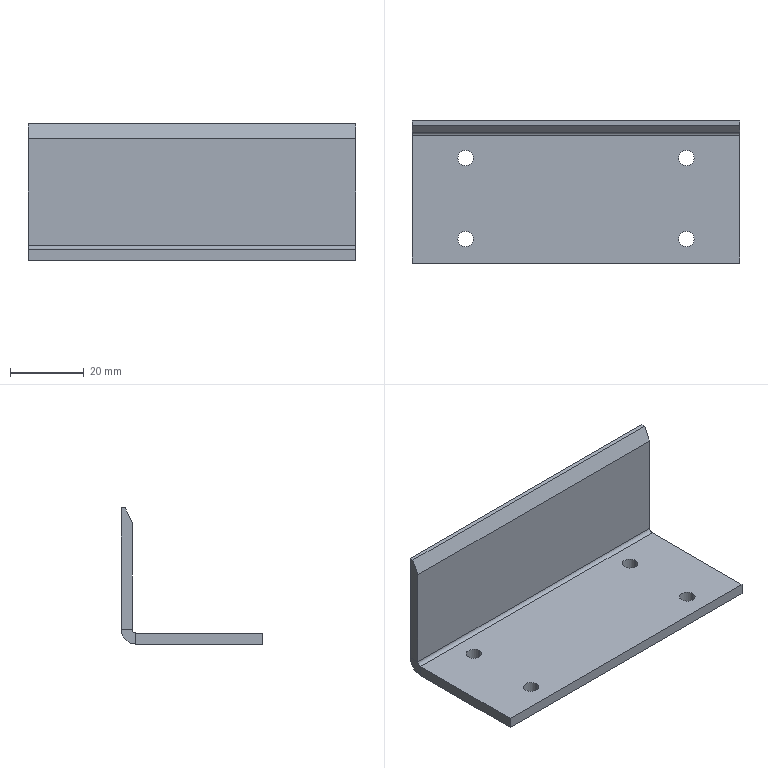Component | SolidWorks | AA-1_TransitionPlate-1 | 1 solid | 23 faces | box 89 x 38.51 x 37 mm | volume 18576 mm3 | plane 13 | cylinder 10 | commonest cylinder face diameters 4.2 x8 2 x1 8 x1
STEP:
#1=COLOUR_RGB('',0.7922,0.8196,0.9333);
#2=FILL_AREA_STYLE_COLOUR('',#1);
#3=FILL_AREA_STYLE('',(#2));
#4=SURFACE_STYLE_FILL_AREA(#3);
#5=SURFACE_SIDE_STYLE('',(#4));
#6=SURFACE_STYLE_USAGE(.BOTH.,#5);
#7=PRESENTATION_STYLE_ASSIGNMENT((#6));
#8=CARTESIAN_POINT('',(-18.558,-12.235,44.862));
#9=VERTEX_POINT('',#8);
#10=CARTESIAN_POINT('',(-18.393,-12.235,44.862));
#11=VERTEX_POINT('',#10);
#12=CARTESIAN_POINT('',(-18.475,-12.235,44.862));
#13=DIRECTION('',(-0.,0.,1.));
#14=DIRECTION('',(1.,0.,0.));
#15=AXIS2_PLACEMENT_3D('',#12,#13,#14);
#16=CIRCLE('',#15,0.08268);
#17=EDGE_CURVE('',#9,#11,#16,.T.);
#18=ORIENTED_EDGE('',*,*,#17,.F.);
#19=CARTESIAN_POINT('',(-18.558,-12.235,44.98));
#20=VERTEX_POINT('',#19);
#21=CARTESIAN_POINT('',(-18.558,-12.235,44.98));
#22=DIRECTION('',(-0.,0.,1.));
#23=VECTOR('',#22,39.37);
#24=LINE('',#21,#23);
#25=EDGE_CURVE('',#9,#20,#24,.T.);
#26=ORIENTED_EDGE('',*,*,#25,.T.);
#27=CARTESIAN_POINT('',(-18.393,-12.235,44.98));
#28=VERTEX_POINT('',#27);
#29=CARTESIAN_POINT('',(-18.475,-12.235,44.98));
#30=DIRECTION('',(-0.,0.,1.));
#31=DIRECTION('',(1.,0.,0.));
#32=AXIS2_PLACEMENT_3D('',#29,#30,#31);
#33=CIRCLE('',#32,0.08268);
#34=EDGE_CURVE('',#20,#28,#33,.T.);
#35=ORIENTED_EDGE('',*,*,#34,.T.);
#36=CARTESIAN_POINT('',(-18.393,-12.235,44.98));
#37=DIRECTION('',(-0.,0.,1.));
#38=VECTOR('',#37,39.37);
#39=LINE('',#36,#38);
#40=EDGE_CURVE('',#11,#28,#39,.T.);
#41=ORIENTED_EDGE('',*,*,#40,.F.);
#42=EDGE_LOOP('',(#18,#26,#35,#41));
#43=FACE_OUTER_BOUND('',#42,.T.);
#44=CARTESIAN_POINT('',(-18.475,-12.235,44.98));
#45=DIRECTION('',(-0.,0.,1.));
#46=DIRECTION('',(1.,0.,0.));
#47=AXIS2_PLACEMENT_3D('',#44,#45,#46);
#48=CYLINDRICAL_SURFACE('',#47,0.08268);
#49=ADVANCED_FACE('',(#43),#48,.F.);
#50=CARTESIAN_POINT('',(-16.196,-12.235,44.862));
#51=VERTEX_POINT('',#50);
#52=CARTESIAN_POINT('',(-16.03,-12.235,44.862));
#53=VERTEX_POINT('',#52);
#54=CARTESIAN_POINT('',(-16.113,-12.235,44.862));
#55=DIRECTION('',(-0.,0.,1.));
#56=DIRECTION('',(1.,0.,0.));
#57=AXIS2_PLACEMENT_3D('',#54,#55,#56);
#58=CIRCLE('',#57,0.08268);
#59=EDGE_CURVE('',#51,#53,#58,.T.);
#60=ORIENTED_EDGE('',*,*,#59,.F.);
#61=CARTESIAN_POINT('',(-16.196,-12.235,44.98));
#62=VERTEX_POINT('',#61);
#63=CARTESIAN_POINT('',(-16.196,-12.235,44.98));
#64=DIRECTION('',(-0.,0.,1.));
#65=VECTOR('',#64,39.37);
#66=LINE('',#63,#65);
#67=EDGE_CURVE('',#51,#62,#66,.T.);
#68=ORIENTED_EDGE('',*,*,#67,.T.);
#69=CARTESIAN_POINT('',(-16.03,-12.235,44.98));
#70=VERTEX_POINT('',#69);
#71=CARTESIAN_POINT('',(-16.113,-12.235,44.98));
#72=DIRECTION('',(-0.,0.,1.));
#73=DIRECTION('',(1.,0.,0.));
#74=AXIS2_PLACEMENT_3D('',#71,#72,#73);
#75=CIRCLE('',#74,0.08268);
#76=EDGE_CURVE('',#62,#70,#75,.T.);
#77=ORIENTED_EDGE('',*,*,#76,.T.);
#78=CARTESIAN_POINT('',(-16.03,-12.235,44.98));
#79=DIRECTION('',(-0.,0.,1.));
#80=VECTOR('',#79,39.37);
#81=LINE('',#78,#80);
#82=EDGE_CURVE('',#53,#70,#81,.T.);
#83=ORIENTED_EDGE('',*,*,#82,.F.);
#84=EDGE_LOOP('',(#60,#68,#77,#83));
#85=FACE_OUTER_BOUND('',#84,.T.);
#86=CARTESIAN_POINT('',(-16.113,-12.235,44.98));
#87=DIRECTION('',(-0.,0.,1.));
#88=DIRECTION('',(1.,0.,0.));
#89=AXIS2_PLACEMENT_3D('',#86,#87,#88);
#90=CYLINDRICAL_SURFACE('',#89,0.08268);
#91=ADVANCED_FACE('',(#85),#90,.F.);
#92=CARTESIAN_POINT('',(-16.196,-13.102,44.862));
#93=VERTEX_POINT('',#92);
#94=CARTESIAN_POINT('',(-16.03,-13.102,44.862));
#95=VERTEX_POINT('',#94);
#96=CARTESIAN_POINT('',(-16.113,-13.102,44.862));
#97=DIRECTION('',(-0.,0.,1.));
#98=DIRECTION('',(1.,0.,0.));
#99=AXIS2_PLACEMENT_3D('',#96,#97,#98);
#100=CIRCLE('',#99,0.08268);
#101=EDGE_CURVE('',#93,#95,#100,.T.);
#102=ORIENTED_EDGE('',*,*,#101,.F.);
#103=CARTESIAN_POINT('',(-16.196,-13.102,44.98));
#104=VERTEX_POINT('',#103);
#105=CARTESIAN_POINT('',(-16.196,-13.102,44.98));
#106=DIRECTION('',(-0.,0.,1.));
#107=VECTOR('',#106,39.37);
#108=LINE('',#105,#107);
#109=EDGE_CURVE('',#93,#104,#108,.T.);
#110=ORIENTED_EDGE('',*,*,#109,.T.);
#111=CARTESIAN_POINT('',(-16.03,-13.102,44.98));
#112=VERTEX_POINT('',#111);
#113=CARTESIAN_POINT('',(-16.113,-13.102,44.98));
#114=DIRECTION('',(-0.,0.,1.));
#115=DIRECTION('',(1.,0.,0.));
#116=AXIS2_PLACEMENT_3D('',#113,#114,#115);
#117=CIRCLE('',#116,0.08268);
#118=EDGE_CURVE('',#104,#112,#117,.T.);
#119=ORIENTED_EDGE('',*,*,#118,.T.);
#120=CARTESIAN_POINT('',(-16.03,-13.102,44.98));
#121=DIRECTION('',(-0.,0.,1.));
#122=VECTOR('',#121,39.37);
#123=LINE('',#120,#122);
#124=EDGE_CURVE('',#95,#112,#123,.T.);
#125=ORIENTED_EDGE('',*,*,#124,.F.);
#126=EDGE_LOOP('',(#102,#110,#119,#125));
#127=FACE_OUTER_BOUND('',#126,.T.);
#128=CARTESIAN_POINT('',(-16.113,-13.102,44.98));
#129=DIRECTION('',(-0.,0.,1.));
#130=DIRECTION('',(1.,0.,0.));
#131=AXIS2_PLACEMENT_3D('',#128,#129,#130);
#132=CYLINDRICAL_SURFACE('',#131,0.08268);
#133=ADVANCED_FACE('',(#127),#132,.F.);
#134=CARTESIAN_POINT('',(-18.558,-13.102,44.862));
#135=VERTEX_POINT('',#134);
#136=CARTESIAN_POINT('',(-18.393,-13.102,44.862));
#137=VERTEX_POINT('',#136);
#138=CARTESIAN_POINT('',(-18.475,-13.102,44.862));
#139=DIRECTION('',(-0.,0.,1.));
#140=DIRECTION('',(1.,0.,0.));
#141=AXIS2_PLACEMENT_3D('',#138,#139,#140);
#142=CIRCLE('',#141,0.08268);
#143=EDGE_CURVE('',#135,#137,#142,.T.);
#144=ORIENTED_EDGE('',*,*,#143,.F.);
#145=CARTESIAN_POINT('',(-18.558,-13.102,44.98));
#146=VERTEX_POINT('',#145);
#147=CARTESIAN_POINT('',(-18.558,-13.102,44.98));
#148=DIRECTION('',(-0.,0.,1.));
#149=VECTOR('',#148,39.37);
#150=LINE('',#147,#149);
#151=EDGE_CURVE('',#135,#146,#150,.T.);
#152=ORIENTED_EDGE('',*,*,#151,.T.);
#153=CARTESIAN_POINT('',(-18.393,-13.102,44.98));
#154=VERTEX_POINT('',#153);
#155=CARTESIAN_POINT('',(-18.475,-13.102,44.98));
#156=DIRECTION('',(-0.,0.,1.));
#157=DIRECTION('',(1.,0.,0.));
#158=AXIS2_PLACEMENT_3D('',#155,#156,#157);
#159=CIRCLE('',#158,0.08268);
#160=EDGE_CURVE('',#146,#154,#159,.T.);
#161=ORIENTED_EDGE('',*,*,#160,.T.);
#162=CARTESIAN_POINT('',(-18.393,-13.102,44.98));
#163=DIRECTION('',(-0.,0.,1.));
#164=VECTOR('',#163,39.37);
#165=LINE('',#162,#164);
#166=EDGE_CURVE('',#137,#154,#165,.T.);
#167=ORIENTED_EDGE('',*,*,#166,.F.);
#168=EDGE_LOOP('',(#144,#152,#161,#167));
#169=FACE_OUTER_BOUND('',#168,.T.);
#170=CARTESIAN_POINT('',(-18.475,-13.102,44.98));
#171=DIRECTION('',(-0.,0.,1.));
#172=DIRECTION('',(1.,0.,0.));
#173=AXIS2_PLACEMENT_3D('',#170,#171,#172);
#174=CYLINDRICAL_SURFACE('',#173,0.08268);
#175=ADVANCED_FACE('',(#169),#174,.F.);
#176=CARTESIAN_POINT('',(-15.542,-11.959,45.02));
#177=VERTEX_POINT('',#176);
#178=CARTESIAN_POINT('',(-15.542,-11.841,45.02));
#179=VERTEX_POINT('',#178);
#180=CARTESIAN_POINT('',(-15.542,-11.959,45.02));
#181=DIRECTION('',(-0.,1.,-0.));
#182=VECTOR('',#181,39.37);
#183=LINE('',#180,#182);
#184=EDGE_CURVE('',#177,#179,#183,.T.);
#185=ORIENTED_EDGE('',*,*,#184,.F.);
#186=CARTESIAN_POINT('',(-15.542,-11.999,44.98));
#187=VERTEX_POINT('',#186);
#188=CARTESIAN_POINT('',(-15.542,-11.999,45.02));
#189=DIRECTION('',(1.,0.,0.));
#190=DIRECTION('',(0.,0.,1.));
#191=AXIS2_PLACEMENT_3D('',#188,#189,#190);
#192=CIRCLE('',#191,0.03937);
#193=EDGE_CURVE('',#187,#177,#192,.T.);
#194=ORIENTED_EDGE('',*,*,#193,.F.);
#195=CARTESIAN_POINT('',(-15.542,-11.999,44.862));
#196=VERTEX_POINT('',#195);
#197=CARTESIAN_POINT('',(-15.542,-11.999,44.862));
#198=DIRECTION('',(-0.,0.,1.));
#199=VECTOR('',#198,39.37);
#200=LINE('',#197,#199);
#201=EDGE_CURVE('',#196,#187,#200,.T.);
#202=ORIENTED_EDGE('',*,*,#201,.F.);
#203=CARTESIAN_POINT('',(-15.542,-11.999,45.02));
#204=DIRECTION('',(1.,0.,0.));
#205=DIRECTION('',(0.,0.,-1.));
#206=AXIS2_PLACEMENT_3D('',#203,#204,#205);
#207=CIRCLE('',#206,0.1575);
#208=EDGE_CURVE('',#196,#179,#207,.T.);
#209=ORIENTED_EDGE('',*,*,#208,.T.);
#210=EDGE_LOOP('',(#185,#194,#202,#209));
#211=FACE_OUTER_BOUND('',#210,.T.);
#212=CARTESIAN_POINT('',(-15.542,-11.959,45.02));
#213=DIRECTION('',(1.,0.,0.));
#214=DIRECTION('',(0.,-0.,-1.));
#215=AXIS2_PLACEMENT_3D('',#212,#213,#214);
#216=PLANE('',#215);
#217=ADVANCED_FACE('',(#211),#216,.T.);
#218=CARTESIAN_POINT('',(-15.542,-11.886,46.319));
#219=VERTEX_POINT('',#218);
#220=CARTESIAN_POINT('',(-15.542,-11.841,46.319));
#221=VERTEX_POINT('',#220);
#222=CARTESIAN_POINT('',(-15.542,-11.959,46.319));
#223=DIRECTION('',(-0.,1.,-0.));
#224=VECTOR('',#223,39.37);
#225=LINE('',#222,#224);
#226=EDGE_CURVE('',#219,#221,#225,.T.);
#227=ORIENTED_EDGE('',*,*,#226,.F.);
#228=CARTESIAN_POINT('',(-15.542,-11.959,46.161));
#229=VERTEX_POINT('',#228);
#230=CARTESIAN_POINT('',(-15.542,-12.464,45.079));
#231=DIRECTION('',(0.,-0.4226,-0.9063));
#232=VECTOR('',#231,39.37);
#233=LINE('',#230,#232);
#234=EDGE_CURVE('',#219,#229,#233,.T.);
#235=ORIENTED_EDGE('',*,*,#234,.T.);
#236=CARTESIAN_POINT('',(-15.542,-11.959,44.98));
#237=DIRECTION('',(-0.,0.,1.));
#238=VECTOR('',#237,39.37);
#239=LINE('',#236,#238);
#240=EDGE_CURVE('',#177,#229,#239,.T.);
#241=ORIENTED_EDGE('',*,*,#240,.F.);
#242=ORIENTED_EDGE('',*,*,#184,.T.);
#243=CARTESIAN_POINT('',(-15.542,-11.841,44.98));
#244=DIRECTION('',(-0.,0.,1.));
#245=VECTOR('',#244,39.37);
#246=LINE('',#243,#245);
#247=EDGE_CURVE('',#179,#221,#246,.T.);
#248=ORIENTED_EDGE('',*,*,#247,.T.);
#249=EDGE_LOOP('',(#227,#235,#241,#242,#248));
#250=FACE_OUTER_BOUND('',#249,.T.);
#251=CARTESIAN_POINT('',(-15.542,-11.999,44.862));
#252=DIRECTION('',(1.,0.,0.));
#253=DIRECTION('',(0.,-0.,-1.));
#254=AXIS2_PLACEMENT_3D('',#251,#252,#253);
#255=PLANE('',#254);
#256=ADVANCED_FACE('',(#250),#255,.T.);
#257=CARTESIAN_POINT('',(-19.046,-11.999,44.98));
#258=VERTEX_POINT('',#257);
#259=CARTESIAN_POINT('',(-19.046,-11.999,44.862));
#260=VERTEX_POINT('',#259);
#261=CARTESIAN_POINT('',(-19.046,-11.999,44.98));
#262=DIRECTION('',(0.,-0.,-1.));
#263=VECTOR('',#262,39.37);
#264=LINE('',#261,#263);
#265=EDGE_CURVE('',#258,#260,#264,.T.);
#266=ORIENTED_EDGE('',*,*,#265,.F.);
#267=CARTESIAN_POINT('',(-19.046,-11.959,45.02));
#268=VERTEX_POINT('',#267);
#269=CARTESIAN_POINT('',(-19.046,-11.999,45.02));
#270=DIRECTION('',(1.,0.,0.));
#271=DIRECTION('',(0.,0.,1.));
#272=AXIS2_PLACEMENT_3D('',#269,#270,#271);
#273=CIRCLE('',#272,0.03937);
#274=EDGE_CURVE('',#258,#268,#273,.T.);
#275=ORIENTED_EDGE('',*,*,#274,.T.);
#276=CARTESIAN_POINT('',(-19.046,-11.841,45.02));
#277=VERTEX_POINT('',#276);
#278=CARTESIAN_POINT('',(-19.046,-11.841,45.02));
#279=DIRECTION('',(0.,-1.,0.));
#280=VECTOR('',#279,39.37);
#281=LINE('',#278,#280);
#282=EDGE_CURVE('',#277,#268,#281,.T.);
#283=ORIENTED_EDGE('',*,*,#282,.F.);
#284=CARTESIAN_POINT('',(-19.046,-11.999,45.02));
#285=DIRECTION('',(1.,0.,0.));
#286=DIRECTION('',(0.,0.,-1.));
#287=AXIS2_PLACEMENT_3D('',#284,#285,#286);
#288=CIRCLE('',#287,0.1575);
#289=EDGE_CURVE('',#260,#277,#288,.T.);
#290=ORIENTED_EDGE('',*,*,#289,.F.);
#291=EDGE_LOOP('',(#266,#275,#283,#290));
#292=FACE_OUTER_BOUND('',#291,.T.);
#293=CARTESIAN_POINT('',(-19.046,-11.999,44.98));
#294=DIRECTION('',(-1.,-0.,-0.));
#295=DIRECTION('',(-0.,0.,1.));
#296=AXIS2_PLACEMENT_3D('',#293,#294,#295);
#297=PLANE('',#296);
#298=ADVANCED_FACE('',(#292),#297,.T.);
#299=CARTESIAN_POINT('',(-19.046,-13.357,44.98));
#300=VERTEX_POINT('',#299);
#301=CARTESIAN_POINT('',(-19.046,-13.357,44.98));
#302=DIRECTION('',(-0.,1.,-0.));
#303=VECTOR('',#302,39.37);
#304=LINE('',#301,#303);
#305=EDGE_CURVE('',#300,#258,#304,.T.);
#306=ORIENTED_EDGE('',*,*,#305,.T.);
#307=ORIENTED_EDGE('',*,*,#265,.T.);
#308=CARTESIAN_POINT('',(-19.046,-13.357,44.862));
#309=VERTEX_POINT('',#308);
#310=CARTESIAN_POINT('',(-19.046,-13.357,44.862));
#311=DIRECTION('',(-0.,1.,-0.));
#312=VECTOR('',#311,39.37);
#313=LINE('',#310,#312);
#314=EDGE_CURVE('',#309,#260,#313,.T.);
#315=ORIENTED_EDGE('',*,*,#314,.F.);
#316=CARTESIAN_POINT('',(-19.046,-13.357,44.862));
#317=DIRECTION('',(-0.,0.,1.));
#318=VECTOR('',#317,39.37);
#319=LINE('',#316,#318);
#320=EDGE_CURVE('',#309,#300,#319,.T.);
#321=ORIENTED_EDGE('',*,*,#320,.T.);
#322=EDGE_LOOP('',(#306,#307,#315,#321));
#323=FACE_OUTER_BOUND('',#322,.T.);
#324=CARTESIAN_POINT('',(-19.046,-11.841,45.02));
#325=DIRECTION('',(-1.,-0.,-0.));
#326=DIRECTION('',(-0.,0.,1.));
#327=AXIS2_PLACEMENT_3D('',#324,#325,#326);
#328=PLANE('',#327);
#329=ADVANCED_FACE('',(#323),#328,.T.);
#330=CARTESIAN_POINT('',(-19.046,-11.841,46.319));
#331=VERTEX_POINT('',#330);
#332=CARTESIAN_POINT('',(-19.046,-11.841,44.98));
#333=DIRECTION('',(-0.,0.,1.));
#334=VECTOR('',#333,39.37);
#335=LINE('',#332,#334);
#336=EDGE_CURVE('',#277,#331,#335,.T.);
#337=ORIENTED_EDGE('',*,*,#336,.T.);
#338=CARTESIAN_POINT('',(-15.542,-11.841,46.319));
#339=DIRECTION('',(-1.,-0.,-0.));
#340=VECTOR('',#339,39.37);
#341=LINE('',#338,#340);
#342=EDGE_CURVE('',#221,#331,#341,.T.);
#343=ORIENTED_EDGE('',*,*,#342,.F.);
#344=ORIENTED_EDGE('',*,*,#247,.F.);
#345=CARTESIAN_POINT('',(-15.542,-11.841,45.02));
#346=DIRECTION('',(-1.,-0.,-0.));
#347=VECTOR('',#346,39.37);
#348=LINE('',#345,#347);
#349=EDGE_CURVE('',#179,#277,#348,.T.);
#350=ORIENTED_EDGE('',*,*,#349,.T.);
#351=EDGE_LOOP('',(#337,#343,#344,#350));
#352=FACE_OUTER_BOUND('',#351,.T.);
#353=CARTESIAN_POINT('',(-15.542,-11.841,44.98));
#354=DIRECTION('',(0.,-1.,0.));
#355=DIRECTION('',(-1.,-0.,-0.));
#356=AXIS2_PLACEMENT_3D('',#353,#354,#355);
#357=PLANE('',#356);
#358=ADVANCED_FACE('',(#352),#357,.F.);
#359=CARTESIAN_POINT('',(-19.046,-11.886,46.319));
#360=VERTEX_POINT('',#359);
#361=CARTESIAN_POINT('',(-19.046,-11.959,46.319));
#362=DIRECTION('',(-0.,1.,-0.));
#363=VECTOR('',#362,39.37);
#364=LINE('',#361,#363);
#365=EDGE_CURVE('',#360,#331,#364,.T.);
#366=ORIENTED_EDGE('',*,*,#365,.F.);
#367=CARTESIAN_POINT('',(-15.542,-11.886,46.319));
#368=DIRECTION('',(1.,0.,0.));
#369=VECTOR('',#368,39.37);
#370=LINE('',#367,#369);
#371=EDGE_CURVE('',#360,#219,#370,.T.);
#372=ORIENTED_EDGE('',*,*,#371,.T.);
#373=ORIENTED_EDGE('',*,*,#226,.T.);
#374=ORIENTED_EDGE('',*,*,#342,.T.);
#375=EDGE_LOOP('',(#366,#372,#373,#374));
#376=FACE_OUTER_BOUND('',#375,.T.);
#377=CARTESIAN_POINT('',(-15.542,-11.959,46.319));
#378=DIRECTION('',(-0.,0.,1.));
#379=DIRECTION('',(1.,0.,0.));
#380=AXIS2_PLACEMENT_3D('',#377,#378,#379);
#381=PLANE('',#380);
#382=ADVANCED_FACE('',(#376),#381,.T.);
#383=ORIENTED_EDGE('',*,*,#240,.T.);
#384=CARTESIAN_POINT('',(-19.046,-11.959,46.161));
#385=VERTEX_POINT('',#384);
#386=CARTESIAN_POINT('',(-15.542,-11.959,46.161));
#387=DIRECTION('',(-1.,-0.,-0.));
#388=VECTOR('',#387,39.37);
#389=LINE('',#386,#388);
#390=EDGE_CURVE('',#229,#385,#389,.T.);
#391=ORIENTED_EDGE('',*,*,#390,.T.);
#392=CARTESIAN_POINT('',(-19.046,-11.959,44.98));
#393=DIRECTION('',(-0.,0.,1.));
#394=VECTOR('',#393,39.37);
#395=LINE('',#392,#394);
#396=EDGE_CURVE('',#268,#385,#395,.T.);
#397=ORIENTED_EDGE('',*,*,#396,.F.);
#398=CARTESIAN_POINT('',(-15.542,-11.959,45.02));
#399=DIRECTION('',(-1.,-0.,-0.));
#400=VECTOR('',#399,39.37);
#401=LINE('',#398,#400);
#402=EDGE_CURVE('',#177,#268,#401,.T.);
#403=ORIENTED_EDGE('',*,*,#402,.F.);
#404=EDGE_LOOP('',(#383,#391,#397,#403));
#405=FACE_OUTER_BOUND('',#404,.T.);
#406=CARTESIAN_POINT('',(-15.542,-11.959,44.98));
#407=DIRECTION('',(0.,-1.,0.));
#408=DIRECTION('',(-1.,-0.,-0.));
#409=AXIS2_PLACEMENT_3D('',#406,#407,#408);
#410=PLANE('',#409);
#411=ADVANCED_FACE('',(#405),#410,.T.);
#412=ORIENTED_EDGE('',*,*,#274,.F.);
#413=CARTESIAN_POINT('',(-15.542,-11.999,44.98));
#414=DIRECTION('',(-1.,-0.,-0.));
#415=VECTOR('',#414,39.37);
#416=LINE('',#413,#415);
#417=EDGE_CURVE('',#187,#258,#416,.T.);
#418=ORIENTED_EDGE('',*,*,#417,.F.);
#419=ORIENTED_EDGE('',*,*,#193,.T.);
#420=ORIENTED_EDGE('',*,*,#402,.T.);
#421=EDGE_LOOP('',(#412,#418,#419,#420));
#422=FACE_OUTER_BOUND('',#421,.T.);
#423=CARTESIAN_POINT('',(-15.542,-11.999,45.02));
#424=DIRECTION('',(-1.,-0.,-0.));
#425=DIRECTION('',(0.,0.,1.));
#426=AXIS2_PLACEMENT_3D('',#423,#424,#425);
#427=CYLINDRICAL_SURFACE('',#426,0.03937);
#428=ADVANCED_FACE('',(#422),#427,.F.);
#429=CARTESIAN_POINT('',(-18.475,-12.235,44.98));
#430=DIRECTION('',(-0.,0.,1.));
#431=DIRECTION('',(1.,0.,0.));
#432=AXIS2_PLACEMENT_3D('',#429,#430,#431);
#433=CIRCLE('',#432,0.08268);
#434=EDGE_CURVE('',#28,#20,#433,.T.);
#435=ORIENTED_EDGE('',*,*,#434,.F.);
#436=ORIENTED_EDGE('',*,*,#34,.F.);
#437=EDGE_LOOP('',(#435,#436));
#438=FACE_BOUND('',#437,.T.);
#439=CARTESIAN_POINT('',(-16.113,-12.235,44.98));
#440=DIRECTION('',(-0.,0.,1.));
#441=DIRECTION('',(1.,0.,0.));
#442=AXIS2_PLACEMENT_3D('',#439,#440,#441);
#443=CIRCLE('',#442,0.08268);
#444=EDGE_CURVE('',#70,#62,#443,.T.);
#445=ORIENTED_EDGE('',*,*,#444,.F.);
#446=ORIENTED_EDGE('',*,*,#76,.F.);
#447=EDGE_LOOP('',(#445,#446));
#448=FACE_BOUND('',#447,.T.);
#449=CARTESIAN_POINT('',(-16.113,-13.102,44.98));
#450=DIRECTION('',(-0.,0.,1.));
#451=DIRECTION('',(1.,0.,0.));
#452=AXIS2_PLACEMENT_3D('',#449,#450,#451);
#453=CIRCLE('',#452,0.08268);
#454=EDGE_CURVE('',#112,#104,#453,.T.);
#455=ORIENTED_EDGE('',*,*,#454,.F.);
#456=ORIENTED_EDGE('',*,*,#118,.F.);
#457=EDGE_LOOP('',(#455,#456));
#458=FACE_BOUND('',#457,.T.);
#459=CARTESIAN_POINT('',(-18.475,-13.102,44.98));
#460=DIRECTION('',(-0.,0.,1.));
#461=DIRECTION('',(1.,0.,0.));
#462=AXIS2_PLACEMENT_3D('',#459,#460,#461);
#463=CIRCLE('',#462,0.08268);
#464=EDGE_CURVE('',#154,#146,#463,.T.);
#465=ORIENTED_EDGE('',*,*,#464,.F.);
#466=ORIENTED_EDGE('',*,*,#160,.F.);
#467=EDGE_LOOP('',(#465,#466));
#468=FACE_BOUND('',#467,.T.);
#469=ORIENTED_EDGE('',*,*,#305,.F.);
#470=CARTESIAN_POINT('',(-15.542,-13.357,44.98));
#471=VERTEX_POINT('',#470);
#472=CARTESIAN_POINT('',(-15.542,-13.357,44.98));
#473=DIRECTION('',(-1.,-0.,-0.));
#474=VECTOR('',#473,39.37);
#475=LINE('',#472,#474);
#476=EDGE_CURVE('',#471,#300,#475,.T.);
#477=ORIENTED_EDGE('',*,*,#476,.F.);
#478=CARTESIAN_POINT('',(-15.542,-13.357,44.98));
#479=DIRECTION('',(-0.,1.,-0.));
#480=VECTOR('',#479,39.37);
#481=LINE('',#478,#480);
#482=EDGE_CURVE('',#471,#187,#481,.T.);
#483=ORIENTED_EDGE('',*,*,#482,.T.);
#484=ORIENTED_EDGE('',*,*,#417,.T.);
#485=EDGE_LOOP('',(#469,#477,#483,#484));
#486=FACE_OUTER_BOUND('',#485,.T.);
#487=CARTESIAN_POINT('',(-15.542,-13.357,44.98));
#488=DIRECTION('',(-0.,0.,1.));
#489=DIRECTION('',(1.,0.,0.));
#490=AXIS2_PLACEMENT_3D('',#487,#488,#489);
#491=PLANE('',#490);
#492=ADVANCED_FACE('',(#438,#448,#458,#468,#486),#491,.T.);
#493=ORIENTED_EDGE('',*,*,#320,.F.);
#494=CARTESIAN_POINT('',(-15.542,-13.357,44.862));
#495=VERTEX_POINT('',#494);
#496=CARTESIAN_POINT('',(-15.542,-13.357,44.862));
#497=DIRECTION('',(-1.,-0.,-0.));
#498=VECTOR('',#497,39.37);
#499=LINE('',#496,#498);
#500=EDGE_CURVE('',#495,#309,#499,.T.);
#501=ORIENTED_EDGE('',*,*,#500,.F.);
#502=CARTESIAN_POINT('',(-15.542,-13.357,44.862));
#503=DIRECTION('',(-0.,0.,1.));
#504=VECTOR('',#503,39.37);
#505=LINE('',#502,#504);
#506=EDGE_CURVE('',#495,#471,#505,.T.);
#507=ORIENTED_EDGE('',*,*,#506,.T.);
#508=ORIENTED_EDGE('',*,*,#476,.T.);
#509=EDGE_LOOP('',(#493,#501,#507,#508));
#510=FACE_OUTER_BOUND('',#509,.T.);
#511=CARTESIAN_POINT('',(-15.542,-13.357,44.862));
#512=DIRECTION('',(0.,-1.,0.));
#513=DIRECTION('',(-1.,-0.,-0.));
#514=AXIS2_PLACEMENT_3D('',#511,#512,#513);
#515=PLANE('',#514);
#516=ADVANCED_FACE('',(#510),#515,.T.);
#517=CARTESIAN_POINT('',(-18.475,-12.235,44.862));
#518=DIRECTION('',(-0.,0.,1.));
#519=DIRECTION('',(1.,0.,0.));
#520=AXIS2_PLACEMENT_3D('',#517,#518,#519);
#521=CIRCLE('',#520,0.08268);
#522=EDGE_CURVE('',#11,#9,#521,.T.);
#523=ORIENTED_EDGE('',*,*,#522,.T.);
#524=ORIENTED_EDGE('',*,*,#17,.T.);
#525=EDGE_LOOP('',(#523,#524));
#526=FACE_BOUND('',#525,.T.);
#527=CARTESIAN_POINT('',(-16.113,-12.235,44.862));
#528=DIRECTION('',(-0.,0.,1.));
#529=DIRECTION('',(1.,0.,0.));
#530=AXIS2_PLACEMENT_3D('',#527,#528,#529);
#531=CIRCLE('',#530,0.08268);
#532=EDGE_CURVE('',#53,#51,#531,.T.);
#533=ORIENTED_EDGE('',*,*,#532,.T.);
#534=ORIENTED_EDGE('',*,*,#59,.T.);
#535=EDGE_LOOP('',(#533,#534));
#536=FACE_BOUND('',#535,.T.);
#537=CARTESIAN_POINT('',(-16.113,-13.102,44.862));
#538=DIRECTION('',(-0.,0.,1.));
#539=DIRECTION('',(1.,0.,0.));
#540=AXIS2_PLACEMENT_3D('',#537,#538,#539);
#541=CIRCLE('',#540,0.08268);
#542=EDGE_CURVE('',#95,#93,#541,.T.);
#543=ORIENTED_EDGE('',*,*,#542,.T.);
#544=ORIENTED_EDGE('',*,*,#101,.T.);
#545=EDGE_LOOP('',(#543,#544));
#546=FACE_BOUND('',#545,.T.);
#547=CARTESIAN_POINT('',(-18.475,-13.102,44.862));
#548=DIRECTION('',(-0.,0.,1.));
#549=DIRECTION('',(1.,0.,0.));
#550=AXIS2_PLACEMENT_3D('',#547,#548,#549);
#551=CIRCLE('',#550,0.08268);
#552=EDGE_CURVE('',#137,#135,#551,.T.);
#553=ORIENTED_EDGE('',*,*,#552,.T.);
#554=ORIENTED_EDGE('',*,*,#143,.T.);
#555=EDGE_LOOP('',(#553,#554));
#556=FACE_BOUND('',#555,.T.);
#557=ORIENTED_EDGE('',*,*,#314,.T.);
#558=CARTESIAN_POINT('',(-15.542,-11.999,44.862));
#559=DIRECTION('',(-1.,-0.,-0.));
#560=VECTOR('',#559,39.37);
#561=LINE('',#558,#560);
#562=EDGE_CURVE('',#196,#260,#561,.T.);
#563=ORIENTED_EDGE('',*,*,#562,.F.);
#564=CARTESIAN_POINT('',(-15.542,-13.357,44.862));
#565=DIRECTION('',(-0.,1.,-0.));
#566=VECTOR('',#565,39.37);
#567=LINE('',#564,#566);
#568=EDGE_CURVE('',#495,#196,#567,.T.);
#569=ORIENTED_EDGE('',*,*,#568,.F.);
#570=ORIENTED_EDGE('',*,*,#500,.T.);
#571=EDGE_LOOP('',(#557,#563,#569,#570));
#572=FACE_OUTER_BOUND('',#571,.T.);
#573=CARTESIAN_POINT('',(-15.542,-13.357,44.862));
#574=DIRECTION('',(-0.,0.,1.));
#575=DIRECTION('',(1.,0.,0.));
#576=AXIS2_PLACEMENT_3D('',#573,#574,#575);
#577=PLANE('',#576);
#578=ADVANCED_FACE('',(#526,#536,#546,#556,#572),#577,.F.);
#579=ORIENTED_EDGE('',*,*,#289,.T.);
#580=ORIENTED_EDGE('',*,*,#349,.F.);
#581=ORIENTED_EDGE('',*,*,#208,.F.);
#582=ORIENTED_EDGE('',*,*,#562,.T.);
#583=EDGE_LOOP('',(#579,#580,#581,#582));
#584=FACE_OUTER_BOUND('',#583,.T.);
#585=CARTESIAN_POINT('',(-15.542,-11.999,45.02));
#586=DIRECTION('',(-1.,-0.,-0.));
#587=DIRECTION('',(0.,0.,1.));
#588=AXIS2_PLACEMENT_3D('',#585,#586,#587);
#589=CYLINDRICAL_SURFACE('',#588,0.1575);
#590=ADVANCED_FACE('',(#584),#589,.T.);
#591=ORIENTED_EDGE('',*,*,#568,.T.);
#592=ORIENTED_EDGE('',*,*,#201,.T.);
#593=ORIENTED_EDGE('',*,*,#482,.F.);
#594=ORIENTED_EDGE('',*,*,#506,.F.);
#595=EDGE_LOOP('',(#591,#592,#593,#594));
#596=FACE_OUTER_BOUND('',#595,.T.);
#597=CARTESIAN_POINT('',(-15.542,-11.999,45.02));
#598=DIRECTION('',(-1.,-0.,-0.));
#599=DIRECTION('',(-0.,0.,1.));
#600=AXIS2_PLACEMENT_3D('',#597,#598,#599);
#601=PLANE('',#600);
#602=ADVANCED_FACE('',(#596),#601,.F.);
#603=ORIENTED_EDGE('',*,*,#396,.T.);
#604=CARTESIAN_POINT('',(-19.046,-12.404,45.209));
#605=DIRECTION('',(-0.,0.4226,0.9063));
#606=VECTOR('',#605,39.37);
#607=LINE('',#604,#606);
#608=EDGE_CURVE('',#385,#360,#607,.T.);
#609=ORIENTED_EDGE('',*,*,#608,.T.);
#610=ORIENTED_EDGE('',*,*,#365,.T.);
#611=ORIENTED_EDGE('',*,*,#336,.F.);
#612=ORIENTED_EDGE('',*,*,#282,.T.);
#613=EDGE_LOOP('',(#603,#609,#610,#611,#612));
#614=FACE_OUTER_BOUND('',#613,.T.);
#615=CARTESIAN_POINT('',(-19.046,-11.999,45.02));
#616=DIRECTION('',(-1.,-0.,-0.));
#617=DIRECTION('',(-0.,0.,1.));
#618=AXIS2_PLACEMENT_3D('',#615,#616,#617);
#619=PLANE('',#618);
#620=ADVANCED_FACE('',(#614),#619,.T.);
#621=ORIENTED_EDGE('',*,*,#234,.F.);
#622=ORIENTED_EDGE('',*,*,#371,.F.);
#623=ORIENTED_EDGE('',*,*,#608,.F.);
#624=ORIENTED_EDGE('',*,*,#390,.F.);
#625=EDGE_LOOP('',(#621,#622,#623,#624));
#626=FACE_OUTER_BOUND('',#625,.T.);
#627=CARTESIAN_POINT('',(-15.542,-11.959,46.161));
#628=DIRECTION('',(0.,0.9063,-0.4226));
#629=DIRECTION('',(-1.,-0.,-0.));
#630=AXIS2_PLACEMENT_3D('',#627,#628,#629);
#631=PLANE('',#630);
#632=ADVANCED_FACE('',(#626),#631,.F.);
#633=ORIENTED_EDGE('',*,*,#151,.F.);
#634=ORIENTED_EDGE('',*,*,#552,.F.);
#635=ORIENTED_EDGE('',*,*,#166,.T.);
#636=ORIENTED_EDGE('',*,*,#464,.T.);
#637=EDGE_LOOP('',(#633,#634,#635,#636));
#638=FACE_OUTER_BOUND('',#637,.T.);
#639=CARTESIAN_POINT('',(-18.475,-13.102,44.98));
#640=DIRECTION('',(-0.,0.,1.));
#641=DIRECTION('',(1.,0.,0.));
#642=AXIS2_PLACEMENT_3D('',#639,#640,#641);
#643=CYLINDRICAL_SURFACE('',#642,0.08268);
#644=ADVANCED_FACE('',(#638),#643,.F.);
#645=ORIENTED_EDGE('',*,*,#109,.F.);
#646=ORIENTED_EDGE('',*,*,#542,.F.);
#647=ORIENTED_EDGE('',*,*,#124,.T.);
#648=ORIENTED_EDGE('',*,*,#454,.T.);
#649=EDGE_LOOP('',(#645,#646,#647,#648));
#650=FACE_OUTER_BOUND('',#649,.T.);
#651=CARTESIAN_POINT('',(-16.113,-13.102,44.98));
#652=DIRECTION('',(-0.,0.,1.));
#653=DIRECTION('',(1.,0.,0.));
#654=AXIS2_PLACEMENT_3D('',#651,#652,#653);
#655=CYLINDRICAL_SURFACE('',#654,0.08268);
#656=ADVANCED_FACE('',(#650),#655,.F.);
#657=ORIENTED_EDGE('',*,*,#67,.F.);
#658=ORIENTED_EDGE('',*,*,#532,.F.);
#659=ORIENTED_EDGE('',*,*,#82,.T.);
#660=ORIENTED_EDGE('',*,*,#444,.T.);
#661=EDGE_LOOP('',(#657,#658,#659,#660));
#662=FACE_OUTER_BOUND('',#661,.T.);
#663=CARTESIAN_POINT('',(-16.113,-12.235,44.98));
#664=DIRECTION('',(-0.,0.,1.));
#665=DIRECTION('',(1.,0.,0.));
#666=AXIS2_PLACEMENT_3D('',#663,#664,#665);
#667=CYLINDRICAL_SURFACE('',#666,0.08268);
#668=ADVANCED_FACE('',(#662),#667,.F.);
#669=ORIENTED_EDGE('',*,*,#25,.F.);
#670=ORIENTED_EDGE('',*,*,#522,.F.);
#671=ORIENTED_EDGE('',*,*,#40,.T.);
#672=ORIENTED_EDGE('',*,*,#434,.T.);
#673=EDGE_LOOP('',(#669,#670,#671,#672));
#674=FACE_OUTER_BOUND('',#673,.T.);
#675=CARTESIAN_POINT('',(-18.475,-12.235,44.98));
#676=DIRECTION('',(-0.,0.,1.));
#677=DIRECTION('',(1.,0.,0.));
#678=AXIS2_PLACEMENT_3D('',#675,#676,#677);
#679=CYLINDRICAL_SURFACE('',#678,0.08268);
#680=ADVANCED_FACE('',(#674),#679,.F.);
#681=CLOSED_SHELL('',(#49,#91,#133,#175,#217,#256,#298,#329,#358,#382,#411,#428,#492,#516,#578,#590,#602,#620,#632,#644,#656,#668,#680));
#682=MANIFOLD_SOLID_BREP('',#681);
#683=STYLED_ITEM('',(#7),#682);
#684=(LENGTH_UNIT()NAMED_UNIT(*)SI_UNIT($,.METRE.));
#685=LENGTH_MEASURE_WITH_UNIT(LENGTH_MEASURE(0.0254),#684);
#686=DIMENSIONAL_EXPONENTS(1.,0.,0.,0.,0.,0.,0.);
#687=(CONVERSION_BASED_UNIT('',#685)LENGTH_UNIT()NAMED_UNIT(#686));
#688=UNCERTAINTY_MEASURE_WITH_UNIT(LENGTH_MEASURE(0.00001),#687,'','');
#689=(NAMED_UNIT(*)PLANE_ANGLE_UNIT()SI_UNIT($,.RADIAN.));
#690=(NAMED_UNIT(*)SI_UNIT($,.STERADIAN.)SOLID_ANGLE_UNIT());
#691=(GEOMETRIC_REPRESENTATION_CONTEXT(3)GLOBAL_UNCERTAINTY_ASSIGNED_CONTEXT((#688))GLOBAL_UNIT_ASSIGNED_CONTEXT((#687,#689,#690))REPRESENTATION_CONTEXT('',''));
#692=MECHANICAL_DESIGN_GEOMETRIC_PRESENTATION_REPRESENTATION('',(#683),#691);
#693=CARTESIAN_POINT('',(0.,0.,0.));
#694=DIRECTION('',(0.,0.,1.));
#695=DIRECTION('',(1.,0.,0.));
#696=AXIS2_PLACEMENT_3D('',#693,#694,#695);
#697=(LENGTH_UNIT()NAMED_UNIT(*)SI_UNIT($,.METRE.));
#698=LENGTH_MEASURE_WITH_UNIT(LENGTH_MEASURE(0.0254),#697);
#699=DIMENSIONAL_EXPONENTS(1.,0.,0.,0.,0.,0.,0.);
#700=(CONVERSION_BASED_UNIT('',#698)LENGTH_UNIT()NAMED_UNIT(#699));
#701=UNCERTAINTY_MEASURE_WITH_UNIT(LENGTH_MEASURE(0.00001),#700,'','');
#702=(NAMED_UNIT(*)PLANE_ANGLE_UNIT()SI_UNIT($,.RADIAN.));
#703=(NAMED_UNIT(*)SI_UNIT($,.STERADIAN.)SOLID_ANGLE_UNIT());
#704=(GEOMETRIC_REPRESENTATION_CONTEXT(3)GLOBAL_UNCERTAINTY_ASSIGNED_CONTEXT((#701))GLOBAL_UNIT_ASSIGNED_CONTEXT((#700,#702,#703))REPRESENTATION_CONTEXT('',''));
#705=ADVANCED_BREP_SHAPE_REPRESENTATION('',(#682,#696),#704);
#706=PRESENTATION_LAYER_ASSIGNMENT('','',(#683));